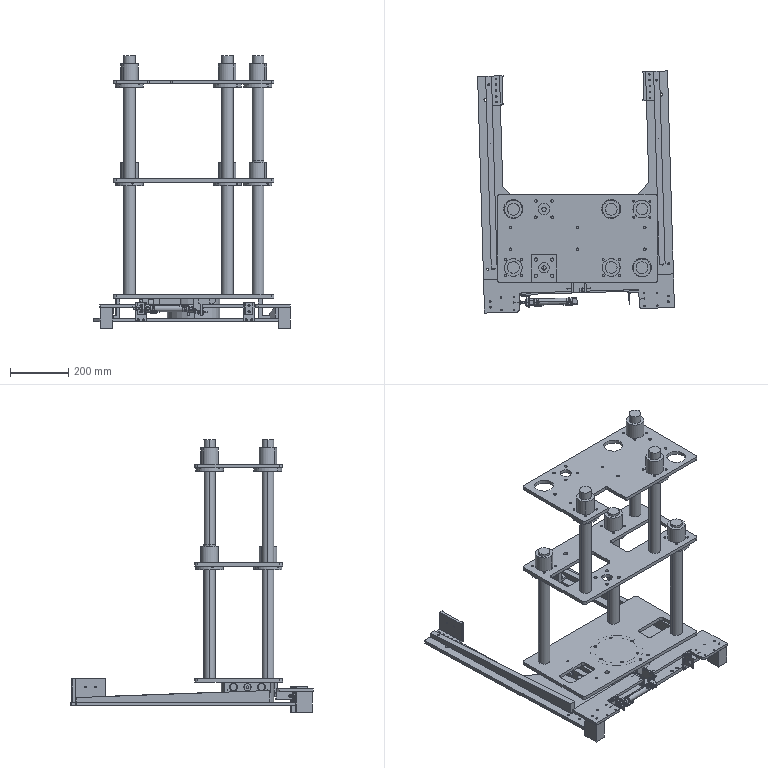Assembly | SolidWorks | mm | 44 component files | 53 solids | 1805 faces | box 673.36 x 828.62 x 932.02 mm | volume 15847557 mm3 | cylinder 923 | plane 540 | cone 190 | torus 114 | sphere 22 | spline 16 | commonest cylinder face diameters 9 x156 6.8 x146 5 x68 10 x50 14 x48 20 x36 5.5 x32 11 x28
Bill of materials:
40Axis | 3 | 45# | Slender solid cylindrical rod with plain flat ends.
40Axis-3 | 3 | 45# | Slender solid cylindrical rod with plain flat ends. Nearly the same as unnamed part but looks slightly thicker for its length.
BearingHousing | 1 | 45# | Short thick-walled ring (annular bushing shape) with an internal step, i.e. a larger bore partway down that meets a smaller bore at a ledge.
BearingPressingCover | 1 | 45# | Flat circular disc with a shallow circular recess in one face and five small through holes: one at the center and four evenly spaced around it.
BufferMAKC1005A | 1 | Standard Parts | Axially symmetric cylindrical body carrying two hexagonal nut-like collars, with stepped diameters at both ends. A thin rod extends from one end and ends in a larger stepped cylindrical tip. Its overall form resembles a plunger-type device.
BufferPad | 2 | 6063 | Rectangular flat plate with three round through holes: two smaller holes near one long edge and one larger hole near a corner on the opposite side.
24OpticalAxis | 2 | 45 | Solid cylinder with an axial hole at one end and a flat or reduced section machined over a short length at the other end.
BrakeBlock | 1 | Industrial Rubber Sheet | Rectangular block with a large circular-arc cutout along one side, forming a concave saddle face. Four radial holes run through the curved face.
CopperSleeve24X27X10 | 2 | Bronze Bronze | Thin-walled cylindrical tube or sleeve, with a length similar to its outer diameter.
CylinderLockingBlock | 1 | Q235 | Rectangular bar with three large round through holes across its wide face and two small holes near the ends running perpendicular to them.
CylinderLockingBlock2 | 1 | 6063 | Rectangular bar with seven round through holes in a single row on its wide face. The hole sizes follow a symmetric pattern: small, large, small, medium, small, large, small.
ClampingCylinderMountingPlate | 1 | 6063 | Two separate, mirror-image, thin L-shaped plates. Each has a wider end region with a pattern of small holes and a rounded inside corner, plus small notches or holes at the narrow end.
CylinderBasePlate2 | 1 | 6063 | Flat rectangular plate with rounded corners, two rounded-rectangle cutouts near the short ends, and a scattered pattern of small through-holes.
CylinderFixingPlate | 1 | 6063 | Flat rectangular plate with rounded corners, a rectangular notch cut into one long edge, several large round openings, and smaller holes, some in four-hole patterns around the openings.
CylinderFixingPlate2 | 2 | 6063 | Small thick rectangular plate with four through-holes: two smaller holes on the centerline and two larger holes side by side near one end. There is a small step along one edge.
CylinderFixingSheetMetal | 2 | Q235 | Bent sheet-style angle bracket with two flanges about 90 degrees apart. One flange has a large round hole and the other has two smaller holes.
CylinderMountingPlate | 2 | 6063 | Thick L-shaped angle block with a vertical wall and a horizontal base flange. The base has a row of five holes and the wall has four holes. There is a small lip or step along the back edge.
CylinderPanel | 1 | 6063 | Flat rectangular plate with rounded corners, two large rounded-rectangle cutouts in the middle band, round openings near the corners with four-hole patterns, and pairs of small holes.
LMF40UU | 6 | Standard Parts | Flanged tubular sleeve: a round tube with a through-bore standing on a wider circular flange that has four through-holes.
MiniCylinderMF20x100SU_0_+_CS1-M-2 | 1 | Standard Parts | Elongated multi-feature body that looks like a compact linear cylinder or actuator: a long cylindrical barrel between two end blocks with side ports, a slender rod with nuts and a stepped tip at one end, and small clip-like attachments on the barrel.
NylonBlock6 | 2 | Nylon 101 | Solid rectangular block with two round holes on one face.
RotatingAxis100 | 1 | 45# | Round cap-like part: a thin circular flange plate on top of a shorter, smaller-diameter cylindrical body. The flange has six evenly spaced small holes.
RotatingPlatform | 1 | 6063 | Large flat U-shaped plate: two long parallel arms joined by a base with angled inner corners. The base has a central large round opening with a ring of small holes around it. There are elongated slots near the arm tips and many small holes.
Stiffener | 2 | 6063 | Long slender bar with a single small hole near one end. Some views suggest a tapered or angled profile.
StopBlock2 | 1 | Q235 | Flat plate of constant thickness with an irregular profile: straight top edge, vertical left edge, concave circular-arc notch at the lower-left corner, sloped bottom edge rising to a short vertical right edge. Two round holes go into the narrow top edge face.
tapered roller bearings gb | 1 |  | Ring-shaped assembly that looks like a roller bearing: an outer ring, an inner ring with a central bore, and a single circle of short cylindrical rollers between them. The inner ring sticks out axially past the outer ring on one face.
thrust ball bearings gb | 1 |  | Thrust-bearing-like stack: two flat annular washers of similar outside diameter, separated by a single ring of spherical balls set around the central axis.
Mates:
1. concentric | ClampingCylinderMountingPlate-1 face at (30.86, -166.128, -1221.21) dir (-0.9996, -0.02918, 0) r 2.5 | BufferPad-1 face at (30.86, -166.128, -1221.21) dir (-0.9996, -0.02918, 0) r 3.5
2. coincident | ClampingCylinderMountingPlate-1 face at (27.795, -61.172, -1226.21) dir (-0.9996, -0.02918, 0) | BufferPad-1 face at (30.422, -151.134, -1233.71) dir (0.9996, 0.02918, 0)
3. parallel | ClampingCylinderMountingPlate-1 face at (180.358, -146.757, -1216.21) dir (0, 0, 1) | BufferPad-1 face at (25.227, -178.798, -1216.21) dir (0, 0, 1)
4. concentric | BufferMAKC1005A-1 face at (24.773, -171.808, -1241.21) dir (-0.9996, -0.02918, 0) r 5 | BufferPad-1 face at (31.02, -171.625, -1241.21) dir (-0.9996, -0.02918, 0) r 5.5
5. coincident | BufferMAKC1005A-1 face at (30.943, -168.982, -1238.343) dir (-0.9996, -0.02918, 0) | BufferPad-1 face at (30.422, -151.134, -1233.71) dir (0.9996, 0.02918, 0)
6. concentric | ClampingCylinderMountingPlate-1 face at (-19.995, -137.6, -1221.21) dir (0.9996, 0.02918, 0) r 2.5 | BufferPad-2 face at (-13.997, -137.425, -1221.21) dir (-0.9996, -0.02918, 0) r 3.5
7. coincident | ClampingCylinderMountingPlate-1 face at (-22.183, -62.632, -1226.21) dir (0.9996, 0.02918, 0) | BufferPad-2 face at (-19.557, -152.593, -1233.71) dir (-0.9996, -0.02918, 0)
8. coincident | BufferPad-1 face at (25.227, -178.798, -1216.21) dir (0, 0, 1) | BufferPad-2 face at (-18.754, -180.082, -1216.21) dir (0, 0, 1)
9. concentric | ClampingCylinderMountingPlate-1 face at (-297.978, -210.743, -1226.21) dir (0, 0, -1) r 3.4 | NylonBlock6-1 face at (-297.978, -210.743, -1296.21) dir (0, 0, -1) r 4.5
10. concentric | ClampingCylinderMountingPlate-1 face at (-297.395, -230.735, -1226.21) dir (0, 0, -1) r 3.4 | NylonBlock6-1 face at (-297.395, -230.735, -1296.21) dir (0, 0, -1) r 7.5
11. coincident | ClampingCylinderMountingPlate-1 face at (-169.493, -156.971, -1226.21) dir (0, 0, -1) | NylonBlock6-1 face at (-297.687, -220.739, -1226.21) dir (0, 0, 1)
12. coincident | MiniCylinderMF20x100SU_0_+_CS1-M-2-1 face at (-165.026, -220.867, -1229.292) dir (0.9996, 0.02918, 0) | CylinderFixingSheetMetal-1 face at (-165.26, -212.871, -1229.21) dir (-0.9996, -0.02918, 0)
13. concentric | MiniCylinderMF20x100SU_0_+_CS1-M-2-1 face at (-81.252, -211.919, -1229.21) dir (0.9996, 0.02918, 0) r 10.7 | CylinderFixingSheetMetal-1 face at (-190.205, -215.1, -1229.21) dir (0.9996, 0.02918, 0) r 11
14. concentric | ClampingCylinderMountingPlate-1 face at (311.762, -192.942, -1226.21) dir (0, 0, -1) r 3.4 | NylonBlock6-2 face at (311.762, -192.942, -1296.21) dir (0, 0, -1) r 7.5
15. concentric | ClampingCylinderMountingPlate-1 face at (312.345, -212.933, -1226.21) dir (0, 0, -1) r 3.4 | NylonBlock6-2 face at (312.345, -212.933, -1296.21) dir (0, 0, -1) r 7.5
16. coincident | ClampingCylinderMountingPlate-1 face at (180.358, -146.757, -1226.21) dir (0, 0, -1) | NylonBlock6-2 face at (312.054, -202.937, -1226.21) dir (0, 0, 1)
17. coincident | RotatingPlatform-1 plane at (-4.636, 192.989, -1268.21) dir (0.9996, 0.02918, 0) | ClampingCylinderMountingPlate-1 plane at (5.433, -151.864, -1216.21) dir (0.9996, 0.02918, 0)
18. coincident | RotatingPlatform-1 face at (331.17, -172.366, -1274.21) dir (0.02918, -0.9996, 0) | CylinderFixingPlate2-1 face at (191.229, -176.452, -1241.71) dir (-0.02918, 0.9996, 0)
19. concentric | RotatingPlatform-1 face at (201.225, -176.16, -1268.21) dir (0.02918, -0.9996, 0) r 2.5 | CylinderFixingPlate2-1 face at (201.196, -175.161, -1268.21) dir (0.02918, -0.9996, 0) r 3.5
20. concentric | RotatingPlatform-1 face at (181.234, -176.744, -1268.21) dir (0.02918, -0.9996, 0) r 2.5 | CylinderFixingPlate2-1 face at (181.204, -175.744, -1268.21) dir (0.02918, -0.9996, 0) r 3.5
21. coincident | CylinderFixingSheetMetal-2 face at (178.751, -180.818, -1229.21) dir (-0.02918, 0.9996, 0) | CylinderFixingPlate2-1 face at (191.346, -180.45, -1241.71) dir (0.02918, -0.9996, 0)
22. concentric | CylinderFixingSheetMetal-2 face at (192.572, -222.433, -1240.21) dir (-0.02918, 0.9996, 0) r 3.5 | CylinderFixingPlate2-1 face at (191.346, -180.45, -1240.21) dir (0.02918, -0.9996, 0) r 2.5
23. concentric | CylinderFixingSheetMetal-2 face at (192.572, -222.433, -1218.21) dir (-0.02918, 0.9996, 0) r 3.5 | CylinderFixingPlate2-1 face at (191.346, -180.45, -1218.21) dir (0.02918, -0.9996, 0) r 2.5
24. concentric | RotatingPlatform-1 face at (-188.609, -187.542, -1268.21) dir (0.02918, -0.9996, 0) r 2.5 | CylinderFixingPlate2-2 face at (-188.638, -186.542, -1268.21) dir (0.02918, -0.9996, 0) r 3.5
25. coincident | RotatingPlatform-1 face at (331.17, -172.366, -1274.21) dir (0.02918, -0.9996, 0) | CylinderFixingPlate2-2 face at (-178.613, -187.25, -1241.71) dir (-0.02918, 0.9996, 0)
26. concentric | RotatingPlatform-1 face at (-188.609, -187.542, -1268.21) dir (0.02918, -0.9996, 0) r 2.5 | CylinderFixingPlate2-2 face at (-188.638, -186.542, -1268.21) dir (0.02918, -0.9996, 0) r 3.5
27. coincident | CylinderFixingSheetMetal-1 face at (-165.902, -190.88, -1229.21) dir (-0.02918, 0.9996, 0) | CylinderFixingPlate2-2 face at (-178.496, -191.248, -1241.71) dir (0.02918, -0.9996, 0)
28. concentric | CylinderFixingSheetMetal-1 face at (-177.271, -233.23, -1240.21) dir (-0.02918, 0.9996, 0) r 3.5 | CylinderFixingPlate2-2 face at (-178.496, -191.248, -1240.21) dir (0.02918, -0.9996, 0) r 2.5
29. concentric | CylinderFixingSheetMetal-1 face at (-177.271, -233.23, -1218.21) dir (-0.02918, 0.9996, 0) r 3.5 | CylinderFixingPlate2-2 face at (-178.496, -191.248, -1218.21) dir (0.02918, -0.9996, 0) r 2.5
30. concentric | tapered roller bearings gb-1 face at (1.785, -26.917, -1200.957) dir (0, 0, 1) r 16 | RotatingAxis100-1 face at (1.785, -26.917, -1200.957) dir (0, 0, -1) r 50
31. coincident | tapered roller bearings gb-1 face at (1.785, -26.917, -1200.957) dir (0, 0, 1) | RotatingAxis100-1 face at (1.785, -26.917, -1200.957) dir (0, 0, -1)
32. concentric | tapered roller bearings gb-1 face at (1.785, -26.917, -1200.957) dir (0, 0, 1) r 32.5 | BearingHousing-1 face at (1.785, -26.917, -1184.21) dir (0, 0, -1) r 90
33. coincident | tapered roller bearings gb-1 face at (-17.802, -51.587, -1219.21) dir (0, 0, -1) | BearingHousing-1 face at (1.785, -26.917, -1219.21) dir (0, 0, 1)
34. concentric | RotatingAxis100-1 face at (1.785, -26.917, -1200.957) dir (0, 0, -1) r 50 | BearingPressingCover-1 face at (1.785, -26.917, -1233.21) dir (0, 0, -1) r 67.5
35. concentric | BearingHousing-1 face at (1.785, -26.917, -1224.21) dir (0, 0, -1) r 67.5 | thrust ball bearings gb-1 face at (1.785, -26.917, -1223.836) dir (0, 0, 1) r 12
36. coincident | BearingHousing-1 face at (1.785, -26.917, -1224.21) dir (0, 0, -1) | thrust ball bearings gb-1 face at (0.4129, -31.725, -1224.21) dir (0, 0, 1)
37. coincident | BearingPressingCover-1 face at (1.785, -26.917, -1233.21) dir (0, 0, 1) | thrust ball bearings gb-1 face at (0.4129, -31.725, -1233.21) dir (0, 0, -1)
38. coincident | CylinderBasePlate2-1 face at (1.785, -26.917, -1190.957) dir (0, 0, -1) | RotatingAxis100-1 face at (1.785, -26.917, -1190.957) dir (0, 0, 1)
39. concentric | CylinderBasePlate2-1 face at (1.785, -26.917, -1190.957) dir (0, 0, -1) r 85 | RotatingAxis100-1 face at (1.785, -26.917, -1190.957) dir (0, 0, -1) r 85
40. concentric | CylinderBasePlate2-1 face at (39.285, 38.035, -1180.957) dir (0, 0, -1) r 4.5 | RotatingAxis100-1 face at (39.285, 38.035, -1190.957) dir (0, 0, 1) r 3.4
41. concentric | RotatingPlatform-1 face at (1.785, -26.917, -1264.21) dir (0, 0, 1) r 90 | BearingHousing-1 face at (1.785, -26.917, -1184.21) dir (0, 0, -1) r 90
42. coincident | RotatingPlatform-1 face at (1.785, -26.917, -1264.21) dir (0, 0, 1) | BearingHousing-1 face at (1.785, -26.917, -1264.21) dir (0, 0, -1)
43. concentric | RotatingAxis100-1 face at (-26.5, 1.367, -1272.957) dir (0, 0, -1) r 2.5 | BearingPressingCover-1 face at (-26.5, 1.367, -1248.21) dir (0, 0, -1) r 3.3
44. coincident | RotatingPlatform-1 face at (-4.636, 192.989, -1262.21) dir (0, 0, 1) | Stiffener-1 face at (-273.7, -99.988, -1262.21) dir (0, 0, -1)
45. concentric | RotatingPlatform-1 face at (-302.081, 529.452, -1274.21) dir (0, 0, -1) r 4.5 | Stiffener-1 face at (-302.081, 529.452, -1262.21) dir (0, 0, -1) r 3.4
46. concentric | RotatingPlatform-1 face at (-284.571, -70.292, -1274.21) dir (0, 0, -1) r 4.5 | Stiffener-1 face at (-284.571, -70.292, -1262.21) dir (0, 0, -1) r 3.4
47. coincident | RotatingPlatform-1 face at (-4.636, 192.989, -1262.21) dir (0, 0, 1) | Stiffener-2 face at (301.055, -83.207, -1262.21) dir (0, 0, -1)
48. concentric | RotatingPlatform-1 face at (272.674, 546.232, -1274.21) dir (0, 0, -1) r 4.5 | Stiffener-2 face at (272.674, 546.232, -1262.21) dir (0, 0, -1) r 3.4
49. concentric | Stiffener-2 face at (290.184, -53.512, -1262.21) dir (0, 0, -1) r 3.4 | RotatingPlatform-1 face at (290.184, -53.512, -1274.21) dir (0, 0, -1) r 4.5
50. coincident | RotatingPlatform-1 face at (219.723, 1074.912, -1262.21) dir (-0.9996, -0.02918, 0) | CylinderMountingPlate-1 face at (235.774, 525.147, -1222.21) dir (0.9996, 0.02918, 0)
51. coincident | RotatingPlatform-1 face at (-4.636, 192.989, -1262.21) dir (0, 0, 1) | CylinderMountingPlate-1 face at (234.314, 575.125, -1262.21) dir (0, 0, -1)
52. coincident | RotatingPlatform-1 face at (309.282, 577.314, -1274.21) dir (-0.02918, 0.9996, 0) | CylinderMountingPlate-1 face at (234.314, 575.125, -1182.21) dir (-0.02918, 0.9996, 0)
53. coincident | Stiffener-1 face at (-283.331, 229.872, -1242.21) dir (0.9996, 0.02918, 0) | CylinderMountingPlate-2 face at (-291.502, 509.753, -1222.21) dir (-0.9996, -0.02918, 0)
54. coincident | RotatingPlatform-1 face at (-4.636, 192.989, -1262.21) dir (0, 0, 1) | CylinderMountingPlate-2 face at (-262.554, 460.576, -1262.21) dir (0, 0, -1)
55. coincident | RotatingPlatform-1 face at (309.282, 577.314, -1274.21) dir (-0.02918, 0.9996, 0) | CylinderMountingPlate-2 face at (-265.473, 560.534, -1182.21) dir (-0.02918, 0.9996, 0)
56. concentric | CylinderBasePlate2-1 face at (-163.215, -96.917, -1180.957) dir (0, 0, 1) r 3.4 | ClampingAssembly-2/CylinderLockingBlock-1 face at (-163.215, -96.917, -1227.957) dir (0, 0, -1) r 7.5
57. coincident | CylinderBasePlate2-1 face at (1.785, 3.083, -1192.957) dir (0, 0, -1) | ClampingAssembly-2/CylinderLockingBlock-1 face at (-153.215, 53.083, -1192.957) dir (0, 0, 1)
58. concentric | CylinderBasePlate2-1 face at (-163.215, 43.083, -1180.957) dir (0, 0, 1) r 3.4 | ClampingAssembly-2/CylinderLockingBlock-1 face at (-163.215, 43.083, -1227.957) dir (0, 0, -1) r 7.5
59. coincident | 40Axis-3-1 face at (-218.215, -96.917, -364.191) dir (0, 0, 1) | 40Axis-3-8 face at (116.785, -96.917, -364.191) dir (0, 0, 1)
60. concentric | RotatingPlatform-1 face at (-168.617, -186.958, -1268.21) dir (0.02918, -0.9996, 0) r 2.5 | CylinderFixingPlate2-2 face at (-168.647, -185.958, -1268.21) dir (0.02918, -0.9996, 0) r 3.5
61. coincident | CylinderFixingPlate-1 face at (1.785, 3.083, -458.966) dir (0, 0, -1) | LMF40UU-13 face at (221.785, 103.083, -458.966) dir (0, 0, 1)
62. concentric | CylinderFixingPlate-1 face at (116.785, -96.917, -458.966) dir (0, 0, 1) r 30.5 | LMF40UU-14 face at (116.785, -96.917, -391.966) dir (0, 0, -1) r 30
63. coincident | CylinderFixingPlate-1 face at (1.785, 3.083, -458.966) dir (0, 0, -1) | LMF40UU-14 face at (116.785, -96.917, -458.966) dir (0, 0, 1)
64. concentric | 40Axis-3-7 face at (221.785, 103.083, -364.191) dir (0, 0, -1) r 20 | LMF40UU-13 face at (221.785, 103.083, -391.966) dir (0, 0, -1) r 20
65. concentric | 40Axis-3-8 face at (116.785, -96.917, -364.191) dir (0, 0, -1) r 20 | LMF40UU-14 face at (116.785, -96.917, -391.966) dir (0, 0, -1) r 20
66. concentric | 40Axis-3-1 face at (-218.215, -96.917, -364.191) dir (0, 0, -1) r 20 | LMF40UU-15 face at (-218.215, -96.917, -391.966) dir (0, 0, -1) r 20
67. coincident | CylinderFixingPlate-1 face at (1.785, 3.083, -458.966) dir (0, 0, -1) | LMF40UU-15 face at (-218.215, -96.917, -458.966) dir (0, 0, 1)
68. coincident | CylinderPanel-1 face at (-273.215, 153.083, -784.191) dir (0, 1, 0) | CylinderFixingPlate-1 face at (-273.215, 153.083, -446.966) dir (0, 1, 0)
69. coincident | CylinderPanel-1 face at (-273.215, 153.083, -784.191) dir (-1, 0, 0) | CylinderFixingPlate-1 face at (-273.215, 153.083, -446.966) dir (-1, 0, 0)
70. coincident | 40Axis-3-7 face at (221.785, 103.083, -784.191) dir (0, 0, -1) | 40Axis-3-8 face at (116.785, -96.917, -784.191) dir (0, 0, -1)
71. coincident | 40Axis-3-1 face at (-218.215, -96.917, -784.191) dir (0, 0, -1) | 40Axis-3-7 face at (221.785, 103.083, -784.191) dir (0, 0, -1)
72. coincident | CylinderPanel-1 face at (1.785, 3.083, -784.191) dir (0, 0, 1) | 40Axis-3-7 face at (221.785, 103.083, -784.191) dir (0, 0, -1)
73. concentric | CylinderFixingPlate-1 face at (-218.215, -96.917, -458.966) dir (0, 0, 1) r 30.5 | LMF40UU-15 face at (-218.215, -96.917, -391.966) dir (0, 0, -1) r 30
74. concentric | CylinderFixingPlate-1 face at (221.785, 103.083, -458.966) dir (0, 0, 1) r 30.5 | LMF40UU-13 face at (221.785, 103.083, -391.966) dir (0, 0, -1) r 30
75. concentric | CylinderPanel-1 face at (221.785, -96.917, -784.191) dir (0, 0, -1) r 30.5 | LMF40UU-16 face at (221.785, -96.917, -729.191) dir (0, 0, -1) r 30
76. coincident | CylinderPanel-1 face at (1.785, 3.083, -796.191) dir (0, 0, -1) | LMF40UU-16 face at (221.785, -96.917, -796.191) dir (0, 0, 1)
77. concentric | CylinderPanel-1 face at (116.785, 103.083, -784.191) dir (0, 0, -1) r 30.5 | LMF40UU-17 face at (116.785, 103.083, -729.191) dir (0, 0, -1) r 30
78. coincident | CylinderPanel-1 face at (1.785, 3.083, -796.191) dir (0, 0, -1) | LMF40UU-17 face at (116.785, 103.083, -796.191) dir (0, 0, 1)
79. concentric | CylinderPanel-1 face at (-218.215, 103.083, -784.191) dir (0, 0, -1) r 30.5 | LMF40UU-18 face at (-218.215, 103.083, -729.191) dir (0, 0, -1) r 30
80. coincident | CylinderPanel-1 face at (1.785, 3.083, -796.191) dir (0, 0, -1) | LMF40UU-18 face at (-218.215, 103.083, -796.191) dir (0, 0, 1)
81. concentric | 40Axis-4 face at (-218.215, 103.083, -720.957) dir (0, 0, -1) r 20 | LMF40UU-18 face at (-218.215, 103.083, -729.191) dir (0, 0, -1) r 20
82. concentric | 40Axis-3 face at (221.785, -96.917, -720.957) dir (0, 0, -1) r 20 | LMF40UU-16 face at (221.785, -96.917, -729.191) dir (0, 0, -1) r 20
83. concentric | 40Axis-5 face at (116.785, 103.083, -720.957) dir (0, 0, -1) r 20 | LMF40UU-17 face at (116.785, 103.083, -729.191) dir (0, 0, -1) r 20
84. coincident | 40Axis-3 edge at (221.785, -96.917, -720.957) dir (0, 0, 1) r 20 | 40Axis-5 face at (116.785, 103.083, -720.957) dir (0, 0, 1)
85. coincident | 40Axis-3 face at (221.785, -96.917, -720.957) dir (0, 0, 1) | 40Axis-4 face at (-218.215, 103.083, -720.957) dir (0, 0, 1)
86. coincident | CylinderPanel-1 face at (-273.215, 153.083, -784.191) dir (0, 1, 0) | CylinderBasePlate2-1 face at (-273.215, 153.083, -1180.957) dir (0, 1, 0)
87. coincident | CylinderPanel-1 face at (-273.215, 153.083, -784.191) dir (-1, 0, 0) | CylinderBasePlate2-1 face at (-273.215, 153.083, -1180.957) dir (-1, 0, 0)
88. coincident | CylinderBasePlate2-1 face at (1.785, 3.083, -1180.957) dir (0, 0, 1) | 40Axis-3 face at (221.785, -96.917, -1180.957) dir (0, 0, -1)
89. concentric | CylinderPanel-1 face at (231.785, 103.083, -784.191) dir (0, 0, -1) r 4.5 | 40Axis-3-7 face at (231.785, 103.083, -784.191) dir (0, 0, -1) r 3.4
90. concentric | CylinderPanel-1 face at (-228.215, -96.917, -784.191) dir (0, 0, -1) r 4.5 | 40Axis-3-1 face at (-228.215, -96.917, -784.191) dir (0, 0, -1) r 3.4
91. concentric | CylinderPanel-1 face at (126.785, -96.917, -784.191) dir (0, 0, -1) r 4.5 | 40Axis-3-8 face at (126.785, -96.917, -784.191) dir (0, 0, -1) r 3.4
92. concentric | CylinderBasePlate2-1 face at (126.785, 103.083, -1192.957) dir (0, 0, 1) r 4.5 | 40Axis-5 face at (126.785, 103.083, -1180.957) dir (0, 0, -1) r 3.4
93. concentric | CylinderBasePlate2-1 face at (231.785, -96.917, -1192.957) dir (0, 0, 1) r 4.5 | 40Axis-3 face at (231.785, -96.917, -1180.957) dir (0, 0, -1) r 3.4
94. concentric | CylinderBasePlate2-1 face at (-208.215, 103.083, -1192.957) dir (0, 0, 1) r 4.5 | 40Axis-4 face at (-208.215, 103.083, -1180.957) dir (0, 0, -1) r 3.4
95. concentric | CylinderBasePlate2-1 face at (57.785, -124.917, -1180.957) dir (0, 0, -1) r 4.5 | StopBlock2-1 face at (57.785, -124.917, -1190.957) dir (0, 0, 1) r 3.4
96. coincident | CylinderBasePlate2-1 face at (78.785, -118.917, -1190.957) dir (0, -1, 0) | StopBlock2-1 face at (1.474, -118.917, -1190.957) dir (0, 1, 0)
97. coincident | CylinderBasePlate2-1 face at (1.785, 3.083, -1190.957) dir (0, 0, -1) | StopBlock2-1 face at (76.096, -130.917, -1190.957) dir (0, 0, 1)
98. concentric | RotatingPlatform-1 face at (-0.5499, 53.049, -1262.21) dir (0, 0, -1) r 4.5 | BearingHousing-1 face at (-0.5499, 53.049, -1264.21) dir (0, 0, -1) r 3.4
99. concentric | 24OpticalAxis-1 face at (-40.25, -48, 0) dir (1, 0, 0) r 12 | CylinderLockingBlock2-1 face at (-58.25, -48, 0) dir (-1, 0, 0) r 9
100. coincident | 24OpticalAxis-2 face at (-40.25, 48, 0) dir (-1, 0, 0) | CylinderLockingBlock2-1 face at (-40.25, 48, 0) dir (1, 0, 0)
101. concentric | 24OpticalAxis-2 face at (-40.25, 48, 0) dir (1, 0, 0) r 12 | CylinderLockingBlock2-1 face at (-58.25, 48, 0) dir (-1, 0, 0) r 9
102. coincident | 24OpticalAxis-2 face at (-40.25, 48, 0) dir (-1, 0, 0) | 24OpticalAxis-1 face at (-40.25, -48, 0) dir (-1, 0, 0)
103. concentric | CopperSleeve24X27X10-1 face at (-1.4, -48, 0) dir (-1, 0, 0) r 12 | 24OpticalAxis-1 face at (-40.25, -48, 0) dir (1, 0, 0) r 12
104. concentric | CylinderLockingBlock-1 face at (-21.4, -48, 0) dir (1, 0, 0) r 13.5 | CopperSleeve24X27X10-1 face at (-1.4, -48, 0) dir (-1, 0, 0) r 13.5
105. coincident | CylinderLockingBlock-1 face at (-1.4, 0, 0) dir (1, 0, 0) | CopperSleeve24X27X10-1 face at (-1.4, -48, 0) dir (1, 0, 0)
106. concentric | CopperSleeve24X27X10-2 face at (-1.4, 48, 0) dir (-1, 0, 0) r 12 | 24OpticalAxis-2 face at (-40.25, 48, 0) dir (1, 0, 0) r 12
107. concentric | CylinderLockingBlock-1 face at (-21.4, 48, 0) dir (1, 0, 0) r 13.5 | CopperSleeve24X27X10-2 face at (-1.4, 48, 0) dir (-1, 0, 0) r 13.5
108. coincident | CylinderLockingBlock-1 face at (-1.4, 0, 0) dir (1, 0, 0) | CopperSleeve24X27X10-2 face at (-1.4, 48, 0) dir (1, 0, 0)
109. concentric | CylinderLockingBlock2-1 face at (-58.25, -65, 0) dir (-1, 0, 0) r 3.4 | BrakeBlock-1 face at (-133.25, -65, 0) dir (-1, 0, 0) r 4.5
110. concentric | CylinderLockingBlock2-1 face at (-58.25, 65, 0) dir (-1, 0, 0) r 3.4 | BrakeBlock-1 face at (-133.25, 65, 0) dir (-1, 0, 0) r 4.5
111. coincident | CylinderLockingBlock2-1 face at (-58.25, 0, 0) dir (-1, 0, 0) | BrakeBlock-1 face at (-58.25, 0, 0) dir (1, 0, 0)